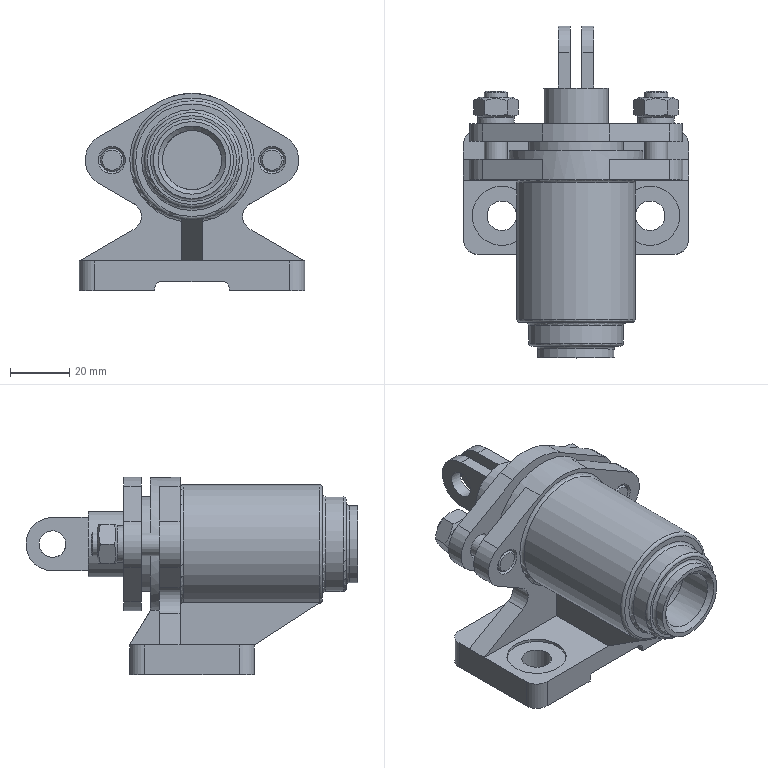Assembly | NX | mm | 11 component files | 11 solids | 155 faces | box 76 x 112 x 66.5 mm | volume 141748 mm3 | plane 85 | cylinder 49 | cone 16 | torus 5 | commonest cylinder face diameters 10 x8 18 x6 32 x4 22 x4 8 x4 9 x4 45 x3 20 x3
Bill of materials:
unnamed part 1 | 2 |  | Hexagonal prism with a central cylindrical through-bore and conical chamfers on both end faces; nut-like shape.
unnamed part 2 | 2 |  | Flat annular ring with rectangular cross-section, cut through by one narrow radial split whose ends are offset axially; looks like a split/helical spring-washer form.
unnamed part 3 | 1 |  | Plain straight cylindrical tube with thin-ish wall and square-cut ends; sleeve or spacer shape.
unnamed part 4 | 2 |  | Solid cylindrical rod with small chamfers on both ends; pin-like shape.
unnamed part 5 | 1 |  | Solid cylindrical body chamfered at one end. The other end has a forked extension: two parallel flat tabs with rounded ends, a slot between them and a common cross-hole through both; clevis-like shape.
unnamed part 6 | 1 |  | Flat annular washer with rectangular section and a chamfer on the outer edge of one face.
unnamed part 7 | 1 |  | Housing/bracket: horizontal cylindrical boss with stepped reduced-diameter end and an axial through-bore, joined to a two-hole oval-type mounting flange at the rear. A perpendicular base foot with one counterbored hole is supported by an angled web/rib; there is a slot below the bore and a recess in the base underside.
unnamed part 8 | 1 |  | Two-hole flange plate with a rounded diamond outline, a central cylindrical spigot/hub on one side and a central through-bore; the two outer lobes each have a round hole.
Mates:
1. fix | pump_body 1 component
2. concentric | bushing 1 arc | pump_body 1 edge
3. concentric | packing 1 edge | pump_body 1 edge
4. concentric | packing 1 edge | packing_gland 1 edge
5. touch align | packing_gland 1 face | pump_body 1 face
6. concentric | spring_washer 2 arc | packing_gland 1 edge
7. concentric | spring_washer 1 arc | packing_gland 1 edge
8. concentric | spring_washer 2 edge | nut 2 arc
9. concentric | stud 2 edge | pump_body 1 edge
10. parallel | nut 2 face | pump_body 1 face
11. concentric | stud 1 edge | pump_body 1 edge
12. concentric | spring_washer 1 edge | nut 1 arc
13. parallel | nut 1 face | pump_body 1 face
14. touch align | plunger 1 face | packing_gland 1 face
15. parallel | plunger 1 face | pump_body 1 face
16. distance | plunger 1 face | packing_gland 1 face